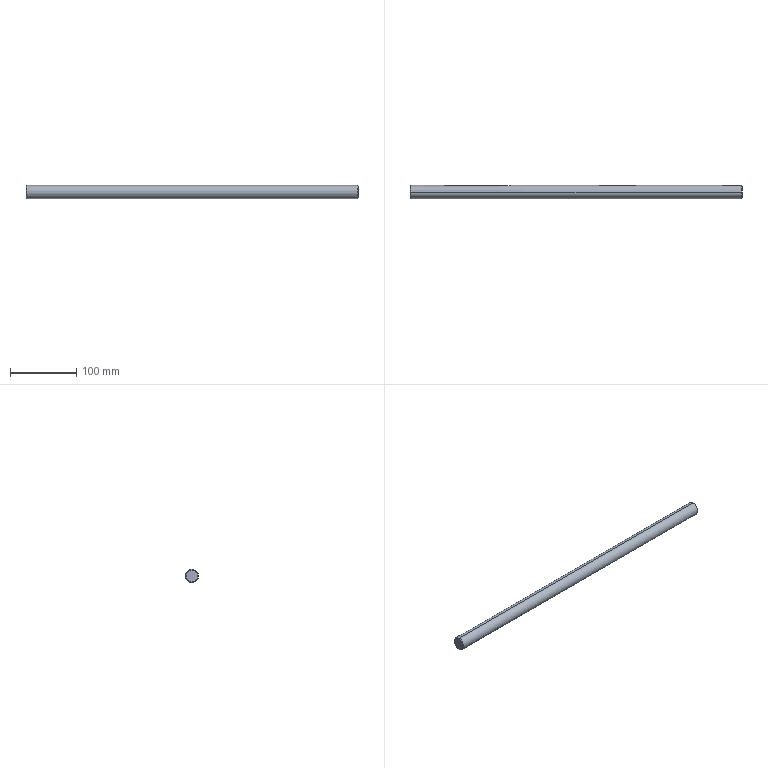Component | SolidWorks | ZL-11-08DriveShaft1-1 | 1 solid | 25 faces | box 503 x 20 x 20 mm | volume 154270 mm3 | plane 11 | cylinder 9 | cone 5 | commonest cylinder face diameters 6 x7 20 x2
build123d program:
from build123d import *

# Parameters (mm, degrees)
SKETCH1_R          = 10
EXTRUDE1_DEPTH     = 251.5
CUT_EXTRUDE1_DEPTH = 3.5
CHAMFER1_SIZE      = 1


with BuildPart() as part:
    # Sketch1 → Extrude1 (new, symmetric)
    with BuildSketch(Plane.XY):
        Circle(SKETCH1_R)
    extrude(amount=EXTRUDE1_DEPTH, both=True)

    # Sketch2 → Cut-Extrude1 (cut)
    with BuildSketch(Plane(origin=(0, 10, 0), x_dir=(-1, 0, 0), z_dir=(0, 1, 0))):
        with BuildLine():
            Line((-3, 251.5), (3, 251.5))
            Line((3, 251.5), (3, 224.5))
            ThreePointArc((3, 224.5), (0, 221.5), (-3, 224.5))
            Line((-3, 224.5), (-3, 251.5))
        make_face()
        with BuildLine():
            Line((-3, -101.5), (-3, -196.5))
            ThreePointArc((-3, -196.5), (0, -199.5), (3, -196.5))
            Line((3, -196.5), (3, -101.5))
            ThreePointArc((3, -101.5), (0, -98.5), (-3, -101.5))
        make_face()
        with BuildLine():
            Line((-3, 88.5), (-3, 38.5))
            ThreePointArc((-3, 38.5), (0, 35.5), (3, 38.5))
            Line((3, 38.5), (3, 88.5))
            ThreePointArc((3, 88.5), (0, 91.5), (-3, 88.5))
        make_face()
    extrude(amount=-CUT_EXTRUDE1_DEPTH, mode=Mode.SUBTRACT)

    # Chamfer1
    chamfer1_edges = [part.edges().sort_by_distance(p)[0] for p in [
        (-10, 0, -251.5),
        (-5.916, -8.062, 251.5),
    ]]
    chamfer(chamfer1_edges, length=CHAMFER1_SIZE)


solid = part.part

# Placed as in the assembly
solid = solid.moved(Location((31.752, 111.22, 0), (0, 90, 0)))
STEP:
#1=COLOUR_RGB('',0.7922,0.8196,0.9333);
#2=FILL_AREA_STYLE_COLOUR('',#1);
#3=FILL_AREA_STYLE('',(#2));
#4=SURFACE_STYLE_FILL_AREA(#3);
#5=SURFACE_SIDE_STYLE('',(#4));
#6=SURFACE_STYLE_USAGE(.BOTH.,#5);
#7=PRESENTATION_STYLE_ASSIGNMENT((#6));
#8=CARTESIAN_POINT('',(-8.651,4.379,0.3543));
#9=VERTEX_POINT('',#8);
#10=CARTESIAN_POINT('',(-8.651,4.379,-0.3543));
#11=VERTEX_POINT('',#10);
#12=CARTESIAN_POINT('',(-8.651,4.379,0.));
#13=DIRECTION('',(-1.,-0.,0.));
#14=DIRECTION('',(0.,0.,-1.));
#15=AXIS2_PLACEMENT_3D('',#12,#13,#14);
#16=CIRCLE('',#15,0.3543);
#17=EDGE_CURVE('',#9,#11,#16,.T.);
#18=ORIENTED_EDGE('',*,*,#17,.F.);
#19=CARTESIAN_POINT('',(-8.612,4.379,0.3937));
#20=VERTEX_POINT('',#19);
#21=CARTESIAN_POINT('',(-8.612,4.379,0.3937));
#22=DIRECTION('',(0.7071,0.,0.7071));
#23=VECTOR('',#22,39.37);
#24=LINE('',#21,#23);
#25=EDGE_CURVE('',#9,#20,#24,.T.);
#26=ORIENTED_EDGE('',*,*,#25,.T.);
#27=CARTESIAN_POINT('',(-8.612,4.379,-0.3937));
#28=VERTEX_POINT('',#27);
#29=CARTESIAN_POINT('',(-8.612,4.379,0.));
#30=DIRECTION('',(1.,0.,-0.));
#31=DIRECTION('',(0.,0.,-1.));
#32=AXIS2_PLACEMENT_3D('',#29,#30,#31);
#33=CIRCLE('',#32,0.3937);
#34=EDGE_CURVE('',#28,#20,#33,.T.);
#35=ORIENTED_EDGE('',*,*,#34,.F.);
#36=CARTESIAN_POINT('',(-8.612,4.379,-0.3937));
#37=DIRECTION('',(0.7071,0.,-0.7071));
#38=VECTOR('',#37,39.37);
#39=LINE('',#36,#38);
#40=EDGE_CURVE('',#11,#28,#39,.T.);
#41=ORIENTED_EDGE('',*,*,#40,.F.);
#42=EDGE_LOOP('',(#18,#26,#35,#41));
#43=FACE_OUTER_BOUND('',#42,.T.);
#44=CARTESIAN_POINT('',(-8.612,4.379,0.));
#45=DIRECTION('',(1.,0.,-0.));
#46=DIRECTION('',(0.,0.,-1.));
#47=AXIS2_PLACEMENT_3D('',#44,#45,#46);
#48=CONICAL_SURFACE('',#47,0.3937,0.7854);
#49=ADVANCED_FACE('',(#43),#48,.T.);
#50=CARTESIAN_POINT('',(11.152,4.379,-0.3543));
#51=VERTEX_POINT('',#50);
#52=CARTESIAN_POINT('',(11.152,4.713,-0.1181));
#53=VERTEX_POINT('',#52);
#54=CARTESIAN_POINT('',(11.152,4.379,0.));
#55=DIRECTION('',(1.,0.,-0.));
#56=DIRECTION('',(0.,0.,-1.));
#57=AXIS2_PLACEMENT_3D('',#54,#55,#56);
#58=CIRCLE('',#57,0.3543);
#59=EDGE_CURVE('',#51,#53,#58,.T.);
#60=ORIENTED_EDGE('',*,*,#59,.F.);
#61=CARTESIAN_POINT('',(11.112,4.379,-0.3937));
#62=VERTEX_POINT('',#61);
#63=CARTESIAN_POINT('',(11.152,4.379,-0.3543));
#64=DIRECTION('',(-0.7071,-0.,-0.7071));
#65=VECTOR('',#64,39.37);
#66=LINE('',#63,#65);
#67=EDGE_CURVE('',#51,#62,#66,.T.);
#68=ORIENTED_EDGE('',*,*,#67,.T.);
#69=CARTESIAN_POINT('',(11.112,4.754,-0.1181));
#70=VERTEX_POINT('',#69);
#71=CARTESIAN_POINT('',(11.112,4.379,0.));
#72=DIRECTION('',(-1.,-0.,0.));
#73=DIRECTION('',(0.,0.,-1.));
#74=AXIS2_PLACEMENT_3D('',#71,#72,#73);
#75=CIRCLE('',#74,0.3937);
#76=EDGE_CURVE('',#70,#62,#75,.T.);
#77=ORIENTED_EDGE('',*,*,#76,.F.);
#78=CARTESIAN_POINT('',(11.152,4.713,-0.1181));
#79=CARTESIAN_POINT('',(11.139,4.727,-0.1181));
#80=CARTESIAN_POINT('',(11.125,4.74,-0.1181));
#81=CARTESIAN_POINT('',(11.112,4.754,-0.1181));
#82=B_SPLINE_CURVE_WITH_KNOTS('',3,(#78,#79,#80,#81),.UNSPECIFIED.,.F.,.F.,(4,4),(0.,0.001453),.UNSPECIFIED.);
#83=EDGE_CURVE('',#53,#70,#82,.T.);
#84=ORIENTED_EDGE('',*,*,#83,.F.);
#85=EDGE_LOOP('',(#60,#68,#77,#84));
#86=FACE_OUTER_BOUND('',#85,.T.);
#87=CARTESIAN_POINT('',(11.152,4.379,0.));
#88=DIRECTION('',(-1.,-0.,0.));
#89=DIRECTION('',(0.,0.,1.));
#90=AXIS2_PLACEMENT_3D('',#87,#88,#89);
#91=CONICAL_SURFACE('',#90,0.3543,0.7854);
#92=ADVANCED_FACE('',(#86),#91,.T.);
#93=ORIENTED_EDGE('',*,*,#67,.F.);
#94=CARTESIAN_POINT('',(11.152,4.379,0.3543));
#95=VERTEX_POINT('',#94);
#96=CARTESIAN_POINT('',(11.152,4.379,0.));
#97=DIRECTION('',(1.,0.,-0.));
#98=DIRECTION('',(0.,0.,-1.));
#99=AXIS2_PLACEMENT_3D('',#96,#97,#98);
#100=CIRCLE('',#99,0.3543);
#101=EDGE_CURVE('',#95,#51,#100,.T.);
#102=ORIENTED_EDGE('',*,*,#101,.F.);
#103=CARTESIAN_POINT('',(11.112,4.379,0.3937));
#104=VERTEX_POINT('',#103);
#105=CARTESIAN_POINT('',(11.152,4.379,0.3543));
#106=DIRECTION('',(-0.7071,-0.,0.7071));
#107=VECTOR('',#106,39.37);
#108=LINE('',#105,#107);
#109=EDGE_CURVE('',#95,#104,#108,.T.);
#110=ORIENTED_EDGE('',*,*,#109,.T.);
#111=CARTESIAN_POINT('',(11.112,4.379,0.));
#112=DIRECTION('',(-1.,-0.,0.));
#113=DIRECTION('',(0.,-0.,-1.));
#114=AXIS2_PLACEMENT_3D('',#111,#112,#113);
#115=CIRCLE('',#114,0.3937);
#116=EDGE_CURVE('',#62,#104,#115,.T.);
#117=ORIENTED_EDGE('',*,*,#116,.F.);
#118=EDGE_LOOP('',(#93,#102,#110,#117));
#119=FACE_OUTER_BOUND('',#118,.T.);
#120=CARTESIAN_POINT('',(11.152,4.379,0.));
#121=DIRECTION('',(-1.,-0.,0.));
#122=DIRECTION('',(0.,0.,1.));
#123=AXIS2_PLACEMENT_3D('',#120,#121,#122);
#124=CONICAL_SURFACE('',#123,0.3543,0.7854);
#125=ADVANCED_FACE('',(#119),#124,.T.);
#126=CARTESIAN_POINT('',(4.852,4.635,0.));
#127=VERTEX_POINT('',#126);
#128=CARTESIAN_POINT('',(4.734,4.635,-0.1181));
#129=VERTEX_POINT('',#128);
#130=CARTESIAN_POINT('',(4.734,4.635,0.));
#131=DIRECTION('',(-0.,1.,-0.));
#132=DIRECTION('',(1.,0.,-0.));
#133=AXIS2_PLACEMENT_3D('',#130,#131,#132);
#134=CIRCLE('',#133,0.1181);
#135=EDGE_CURVE('',#127,#129,#134,.T.);
#136=ORIENTED_EDGE('',*,*,#135,.F.);
#137=CARTESIAN_POINT('',(4.852,4.772,0.));
#138=VERTEX_POINT('',#137);
#139=CARTESIAN_POINT('',(4.852,4.635,0.));
#140=DIRECTION('',(-0.,1.,-0.));
#141=VECTOR('',#140,39.37);
#142=LINE('',#139,#141);
#143=EDGE_CURVE('',#127,#138,#142,.T.);
#144=ORIENTED_EDGE('',*,*,#143,.T.);
#145=CARTESIAN_POINT('',(4.734,4.754,-0.1181));
#146=VERTEX_POINT('',#145);
#147=CARTESIAN_POINT('',(4.734,4.754,-0.1181));
#148=CARTESIAN_POINT('',(4.742,4.754,-0.1181));
#149=CARTESIAN_POINT('',(4.75,4.755,-0.1173));
#150=CARTESIAN_POINT('',(4.765,4.755,-0.1143));
#151=CARTESIAN_POINT('',(4.773,4.756,-0.112));
#152=CARTESIAN_POINT('',(4.794,4.759,-0.1031));
#153=CARTESIAN_POINT('',(4.807,4.761,-0.09437));
#154=CARTESIAN_POINT('',(4.823,4.765,-0.07814));
#155=CARTESIAN_POINT('',(4.828,4.766,-0.07211));
#156=CARTESIAN_POINT('',(4.837,4.768,-0.05931));
#157=CARTESIAN_POINT('',(4.84,4.769,-0.05255));
#158=CARTESIAN_POINT('',(4.846,4.771,-0.03831));
#159=CARTESIAN_POINT('',(4.849,4.771,-0.03076));
#160=CARTESIAN_POINT('',(4.852,4.772,-0.01557));
#161=CARTESIAN_POINT('',(4.852,4.772,-0.00785));
#162=CARTESIAN_POINT('',(4.852,4.772,0.));
#163=B_SPLINE_CURVE_WITH_KNOTS('',3,(#147,#148,#149,#150,#151,#152,#153,#154,#155,#156,#157,#158,#159,#160,#161,#162),.UNSPECIFIED.,.F.,.F.,(4,2,2,2,2,2,2,4),(0.01415,0.01474,0.01533,0.01651,0.0171,0.01769,0.01828,0.01887),.UNSPECIFIED.);
#164=EDGE_CURVE('',#146,#138,#163,.T.);
#165=ORIENTED_EDGE('',*,*,#164,.F.);
#166=CARTESIAN_POINT('',(4.734,4.635,-0.1181));
#167=DIRECTION('',(-0.,1.,-0.));
#168=VECTOR('',#167,39.37);
#169=LINE('',#166,#168);
#170=EDGE_CURVE('',#129,#146,#169,.T.);
#171=ORIENTED_EDGE('',*,*,#170,.F.);
#172=EDGE_LOOP('',(#136,#144,#165,#171));
#173=FACE_OUTER_BOUND('',#172,.T.);
#174=CARTESIAN_POINT('',(4.734,4.635,0.));
#175=DIRECTION('',(-0.,1.,-0.));
#176=DIRECTION('',(1.,0.,-0.));
#177=AXIS2_PLACEMENT_3D('',#174,#175,#176);
#178=CYLINDRICAL_SURFACE('',#177,0.1181);
#179=ADVANCED_FACE('',(#173),#178,.F.);
#180=CARTESIAN_POINT('',(-2.628,4.635,0.));
#181=VERTEX_POINT('',#180);
#182=CARTESIAN_POINT('',(-2.746,4.635,-0.1181));
#183=VERTEX_POINT('',#182);
#184=CARTESIAN_POINT('',(-2.746,4.635,0.));
#185=DIRECTION('',(-0.,1.,-0.));
#186=DIRECTION('',(1.,0.,-0.));
#187=AXIS2_PLACEMENT_3D('',#184,#185,#186);
#188=CIRCLE('',#187,0.1181);
#189=EDGE_CURVE('',#181,#183,#188,.T.);
#190=ORIENTED_EDGE('',*,*,#189,.F.);
#191=CARTESIAN_POINT('',(-2.628,4.772,0.));
#192=VERTEX_POINT('',#191);
#193=CARTESIAN_POINT('',(-2.628,4.635,0.));
#194=DIRECTION('',(-0.,1.,-0.));
#195=VECTOR('',#194,39.37);
#196=LINE('',#193,#195);
#197=EDGE_CURVE('',#181,#192,#196,.T.);
#198=ORIENTED_EDGE('',*,*,#197,.T.);
#199=CARTESIAN_POINT('',(-2.746,4.754,-0.1181));
#200=VERTEX_POINT('',#199);
#201=CARTESIAN_POINT('',(-2.746,4.754,-0.1181));
#202=CARTESIAN_POINT('',(-2.738,4.754,-0.1181));
#203=CARTESIAN_POINT('',(-2.731,4.755,-0.1173));
#204=CARTESIAN_POINT('',(-2.715,4.755,-0.1143));
#205=CARTESIAN_POINT('',(-2.708,4.756,-0.112));
#206=CARTESIAN_POINT('',(-2.686,4.759,-0.1031));
#207=CARTESIAN_POINT('',(-2.673,4.761,-0.09437));
#208=CARTESIAN_POINT('',(-2.657,4.765,-0.07814));
#209=CARTESIAN_POINT('',(-2.652,4.766,-0.07211));
#210=CARTESIAN_POINT('',(-2.644,4.768,-0.05931));
#211=CARTESIAN_POINT('',(-2.64,4.769,-0.05255));
#212=CARTESIAN_POINT('',(-2.634,4.771,-0.03831));
#213=CARTESIAN_POINT('',(-2.632,4.771,-0.03076));
#214=CARTESIAN_POINT('',(-2.629,4.772,-0.01557));
#215=CARTESIAN_POINT('',(-2.628,4.772,-0.00785));
#216=CARTESIAN_POINT('',(-2.628,4.772,0.));
#217=B_SPLINE_CURVE_WITH_KNOTS('',3,(#201,#202,#203,#204,#205,#206,#207,#208,#209,#210,#211,#212,#213,#214,#215,#216),.UNSPECIFIED.,.F.,.F.,(4,2,2,2,2,2,2,4),(0.01415,0.01474,0.01533,0.01651,0.0171,0.01769,0.01828,0.01887),.UNSPECIFIED.);
#218=EDGE_CURVE('',#200,#192,#217,.T.);
#219=ORIENTED_EDGE('',*,*,#218,.F.);
#220=CARTESIAN_POINT('',(-2.746,4.635,-0.1181));
#221=DIRECTION('',(-0.,1.,-0.));
#222=VECTOR('',#221,39.37);
#223=LINE('',#220,#222);
#224=EDGE_CURVE('',#183,#200,#223,.T.);
#225=ORIENTED_EDGE('',*,*,#224,.F.);
#226=EDGE_LOOP('',(#190,#198,#219,#225));
#227=FACE_OUTER_BOUND('',#226,.T.);
#228=CARTESIAN_POINT('',(-2.746,4.635,0.));
#229=DIRECTION('',(-0.,1.,-0.));
#230=DIRECTION('',(1.,0.,-0.));
#231=AXIS2_PLACEMENT_3D('',#228,#229,#230);
#232=CYLINDRICAL_SURFACE('',#231,0.1181);
#233=ADVANCED_FACE('',(#227),#232,.F.);
#234=ORIENTED_EDGE('',*,*,#164,.T.);
#235=CARTESIAN_POINT('',(4.734,4.754,0.1181));
#236=VERTEX_POINT('',#235);
#237=CARTESIAN_POINT('',(4.852,4.772,0.));
#238=CARTESIAN_POINT('',(4.852,4.772,0.007855));
#239=CARTESIAN_POINT('',(4.852,4.772,0.01557));
#240=CARTESIAN_POINT('',(4.849,4.771,0.03073));
#241=CARTESIAN_POINT('',(4.846,4.771,0.03826));
#242=CARTESIAN_POINT('',(4.84,4.769,0.05255));
#243=CARTESIAN_POINT('',(4.837,4.768,0.05932));
#244=CARTESIAN_POINT('',(4.828,4.766,0.07213));
#245=CARTESIAN_POINT('',(4.823,4.765,0.07815));
#246=CARTESIAN_POINT('',(4.807,4.761,0.09439));
#247=CARTESIAN_POINT('',(4.794,4.759,0.1032));
#248=CARTESIAN_POINT('',(4.773,4.756,0.112));
#249=CARTESIAN_POINT('',(4.765,4.755,0.1143));
#250=CARTESIAN_POINT('',(4.75,4.755,0.1174));
#251=CARTESIAN_POINT('',(4.742,4.754,0.1181));
#252=CARTESIAN_POINT('',(4.734,4.754,0.1181));
#253=B_SPLINE_CURVE_WITH_KNOTS('',3,(#237,#238,#239,#240,#241,#242,#243,#244,#245,#246,#247,#248,#249,#250,#251,#252),.UNSPECIFIED.,.F.,.F.,(4,2,2,2,2,2,2,4),(0.,0.0005898,0.00118,0.001769,0.002359,0.003539,0.004129,0.004718),.UNSPECIFIED.);
#254=EDGE_CURVE('',#138,#236,#253,.T.);
#255=ORIENTED_EDGE('',*,*,#254,.T.);
#256=CARTESIAN_POINT('',(2.766,4.754,0.1181));
#257=VERTEX_POINT('',#256);
#258=CARTESIAN_POINT('',(11.152,4.754,0.1181));
#259=DIRECTION('',(-1.,-0.,0.));
#260=VECTOR('',#259,39.37);
#261=LINE('',#258,#260);
#262=EDGE_CURVE('',#236,#257,#261,.T.);
#263=ORIENTED_EDGE('',*,*,#262,.T.);
#264=CARTESIAN_POINT('',(2.766,4.754,-0.1181));
#265=VERTEX_POINT('',#264);
#266=CARTESIAN_POINT('',(2.766,4.754,0.1181));
#267=CARTESIAN_POINT('',(2.758,4.754,0.1181));
#268=CARTESIAN_POINT('',(2.75,4.755,0.1173));
#269=CARTESIAN_POINT('',(2.735,4.755,0.1143));
#270=CARTESIAN_POINT('',(2.728,4.756,0.112));
#271=CARTESIAN_POINT('',(2.713,4.758,0.1061));
#272=CARTESIAN_POINT('',(2.706,4.759,0.1024));
#273=CARTESIAN_POINT('',(2.694,4.761,0.09385));
#274=CARTESIAN_POINT('',(2.688,4.762,0.08892));
#275=CARTESIAN_POINT('',(2.677,4.765,0.07802));
#276=CARTESIAN_POINT('',(2.672,4.766,0.0721));
#277=CARTESIAN_POINT('',(2.663,4.768,0.05934));
#278=CARTESIAN_POINT('',(2.66,4.769,0.05242));
#279=CARTESIAN_POINT('',(2.654,4.771,0.03819));
#280=CARTESIAN_POINT('',(2.652,4.771,0.03082));
#281=CARTESIAN_POINT('',(2.648,4.772,0.01556));
#282=CARTESIAN_POINT('',(2.648,4.772,0.007729));
#283=CARTESIAN_POINT('',(2.648,4.772,-0.007742));
#284=CARTESIAN_POINT('',(2.648,4.772,-0.0155));
#285=CARTESIAN_POINT('',(2.652,4.771,-0.03083));
#286=CARTESIAN_POINT('',(2.654,4.771,-0.03822));
#287=CARTESIAN_POINT('',(2.66,4.769,-0.05246));
#288=CARTESIAN_POINT('',(2.663,4.768,-0.05937));
#289=CARTESIAN_POINT('',(2.672,4.766,-0.07215));
#290=CARTESIAN_POINT('',(2.677,4.765,-0.07806));
#291=CARTESIAN_POINT('',(2.688,4.762,-0.08896));
#292=CARTESIAN_POINT('',(2.694,4.761,-0.09389));
#293=CARTESIAN_POINT('',(2.706,4.759,-0.1024));
#294=CARTESIAN_POINT('',(2.713,4.758,-0.1061));
#295=CARTESIAN_POINT('',(2.728,4.756,-0.112));
#296=CARTESIAN_POINT('',(2.735,4.755,-0.1143));
#297=CARTESIAN_POINT('',(2.75,4.755,-0.1173));
#298=CARTESIAN_POINT('',(2.758,4.754,-0.1181));
#299=CARTESIAN_POINT('',(2.766,4.754,-0.1181));
#300=B_SPLINE_CURVE_WITH_KNOTS('',3,(#266,#267,#268,#269,#270,#271,#272,#273,#274,#275,#276,#277,#278,#279,#280,#281,#282,#283,#284,#285,#286,#287,#288,#289,#290,#291,#292,#293,#294,#295,#296,#297,#298,#299),.UNSPECIFIED.,.F.,.F.,(4,2,2,2,2,2,2,2,2,2,2,2,2,2,2,2,4),(0.004718,0.005308,0.005897,0.006487,0.007076,0.007666,0.008255,0.008845,0.009434,0.01002,0.01061,0.0112,0.01179,0.01238,0.01297,0.01356,0.01415),.UNSPECIFIED.);
#301=EDGE_CURVE('',#257,#265,#300,.T.);
#302=ORIENTED_EDGE('',*,*,#301,.T.);
#303=CARTESIAN_POINT('',(11.152,4.754,-0.1181));
#304=DIRECTION('',(1.,0.,-0.));
#305=VECTOR('',#304,39.37);
#306=LINE('',#303,#305);
#307=EDGE_CURVE('',#265,#146,#306,.T.);
#308=ORIENTED_EDGE('',*,*,#307,.T.);
#309=EDGE_LOOP('',(#234,#255,#263,#302,#308));
#310=FACE_BOUND('',#309,.T.);
#311=ORIENTED_EDGE('',*,*,#218,.T.);
#312=CARTESIAN_POINT('',(-2.746,4.754,0.1181));
#313=VERTEX_POINT('',#312);
#314=CARTESIAN_POINT('',(-2.628,4.772,0.));
#315=CARTESIAN_POINT('',(-2.628,4.772,0.007855));
#316=CARTESIAN_POINT('',(-2.629,4.772,0.01557));
#317=CARTESIAN_POINT('',(-2.632,4.771,0.03073));
#318=CARTESIAN_POINT('',(-2.634,4.771,0.03826));
#319=CARTESIAN_POINT('',(-2.64,4.769,0.05255));
#320=CARTESIAN_POINT('',(-2.644,4.768,0.05932));
#321=CARTESIAN_POINT('',(-2.652,4.766,0.07213));
#322=CARTESIAN_POINT('',(-2.657,4.765,0.07815));
#323=CARTESIAN_POINT('',(-2.673,4.761,0.09439));
#324=CARTESIAN_POINT('',(-2.686,4.759,0.1032));
#325=CARTESIAN_POINT('',(-2.708,4.756,0.112));
#326=CARTESIAN_POINT('',(-2.715,4.755,0.1143));
#327=CARTESIAN_POINT('',(-2.731,4.755,0.1174));
#328=CARTESIAN_POINT('',(-2.738,4.754,0.1181));
#329=CARTESIAN_POINT('',(-2.746,4.754,0.1181));
#330=B_SPLINE_CURVE_WITH_KNOTS('',3,(#314,#315,#316,#317,#318,#319,#320,#321,#322,#323,#324,#325,#326,#327,#328,#329),.UNSPECIFIED.,.F.,.F.,(4,2,2,2,2,2,2,4),(0.,0.0005898,0.00118,0.001769,0.002359,0.003539,0.004129,0.004718),.UNSPECIFIED.);
#331=EDGE_CURVE('',#192,#313,#330,.T.);
#332=ORIENTED_EDGE('',*,*,#331,.T.);
#333=CARTESIAN_POINT('',(-6.486,4.754,0.1181));
#334=VERTEX_POINT('',#333);
#335=CARTESIAN_POINT('',(11.152,4.754,0.1181));
#336=DIRECTION('',(-1.,-0.,0.));
#337=VECTOR('',#336,39.37);
#338=LINE('',#335,#337);
#339=EDGE_CURVE('',#313,#334,#338,.T.);
#340=ORIENTED_EDGE('',*,*,#339,.T.);
#341=CARTESIAN_POINT('',(-6.486,4.754,-0.1181));
#342=VERTEX_POINT('',#341);
#343=CARTESIAN_POINT('',(-6.486,4.754,0.1181));
#344=CARTESIAN_POINT('',(-6.494,4.754,0.1181));
#345=CARTESIAN_POINT('',(-6.502,4.755,0.1173));
#346=CARTESIAN_POINT('',(-6.517,4.755,0.1143));
#347=CARTESIAN_POINT('',(-6.524,4.756,0.112));
#348=CARTESIAN_POINT('',(-6.539,4.758,0.1061));
#349=CARTESIAN_POINT('',(-6.546,4.759,0.1024));
#350=CARTESIAN_POINT('',(-6.558,4.761,0.09385));
#351=CARTESIAN_POINT('',(-6.564,4.762,0.08892));
#352=CARTESIAN_POINT('',(-6.575,4.765,0.07802));
#353=CARTESIAN_POINT('',(-6.58,4.766,0.0721));
#354=CARTESIAN_POINT('',(-6.589,4.768,0.05934));
#355=CARTESIAN_POINT('',(-6.592,4.769,0.05242));
#356=CARTESIAN_POINT('',(-6.598,4.771,0.03819));
#357=CARTESIAN_POINT('',(-6.6,4.771,0.03082));
#358=CARTESIAN_POINT('',(-6.603,4.772,0.01556));
#359=CARTESIAN_POINT('',(-6.604,4.772,0.007729));
#360=CARTESIAN_POINT('',(-6.604,4.772,-0.007742));
#361=CARTESIAN_POINT('',(-6.603,4.772,-0.0155));
#362=CARTESIAN_POINT('',(-6.6,4.771,-0.03083));
#363=CARTESIAN_POINT('',(-6.598,4.771,-0.03822));
#364=CARTESIAN_POINT('',(-6.592,4.769,-0.05246));
#365=CARTESIAN_POINT('',(-6.589,4.768,-0.05937));
#366=CARTESIAN_POINT('',(-6.58,4.766,-0.07215));
#367=CARTESIAN_POINT('',(-6.575,4.765,-0.07806));
#368=CARTESIAN_POINT('',(-6.564,4.762,-0.08896));
#369=CARTESIAN_POINT('',(-6.558,4.761,-0.09389));
#370=CARTESIAN_POINT('',(-6.545,4.759,-0.1024));
#371=CARTESIAN_POINT('',(-6.539,4.758,-0.1061));
#372=CARTESIAN_POINT('',(-6.524,4.756,-0.112));
#373=CARTESIAN_POINT('',(-6.517,4.755,-0.1143));
#374=CARTESIAN_POINT('',(-6.502,4.755,-0.1173));
#375=CARTESIAN_POINT('',(-6.494,4.754,-0.1181));
#376=CARTESIAN_POINT('',(-6.486,4.754,-0.1181));
#377=B_SPLINE_CURVE_WITH_KNOTS('',3,(#343,#344,#345,#346,#347,#348,#349,#350,#351,#352,#353,#354,#355,#356,#357,#358,#359,#360,#361,#362,#363,#364,#365,#366,#367,#368,#369,#370,#371,#372,#373,#374,#375,#376),.UNSPECIFIED.,.F.,.F.,(4,2,2,2,2,2,2,2,2,2,2,2,2,2,2,2,4),(0.004718,0.005308,0.005897,0.006487,0.007076,0.007666,0.008255,0.008845,0.009434,0.01002,0.01061,0.0112,0.01179,0.01238,0.01297,0.01356,0.01415),.UNSPECIFIED.);
#378=EDGE_CURVE('',#334,#342,#377,.T.);
#379=ORIENTED_EDGE('',*,*,#378,.T.);
#380=CARTESIAN_POINT('',(11.152,4.754,-0.1181));
#381=DIRECTION('',(1.,0.,-0.));
#382=VECTOR('',#381,39.37);
#383=LINE('',#380,#382);
#384=EDGE_CURVE('',#342,#200,#383,.T.);
#385=ORIENTED_EDGE('',*,*,#384,.T.);
#386=EDGE_LOOP('',(#311,#332,#340,#379,#385));
#387=FACE_BOUND('',#386,.T.);
#388=ORIENTED_EDGE('',*,*,#76,.T.);
#389=CARTESIAN_POINT('',(11.152,4.379,-0.3937));
#390=DIRECTION('',(-1.,-0.,0.));
#391=VECTOR('',#390,39.37);
#392=LINE('',#389,#391);
#393=EDGE_CURVE('',#62,#28,#392,.T.);
#394=ORIENTED_EDGE('',*,*,#393,.T.);
#395=ORIENTED_EDGE('',*,*,#34,.T.);
#396=CARTESIAN_POINT('',(11.152,4.379,0.3937));
#397=DIRECTION('',(-1.,-0.,0.));
#398=VECTOR('',#397,39.37);
#399=LINE('',#396,#398);
#400=EDGE_CURVE('',#104,#20,#399,.T.);
#401=ORIENTED_EDGE('',*,*,#400,.F.);
#402=CARTESIAN_POINT('',(11.112,4.754,0.1181));
#403=VERTEX_POINT('',#402);
#404=CARTESIAN_POINT('',(11.112,4.379,0.));
#405=DIRECTION('',(-1.,-0.,0.));
#406=DIRECTION('',(0.,0.,-1.));
#407=AXIS2_PLACEMENT_3D('',#404,#405,#406);
#408=CIRCLE('',#407,0.3937);
#409=EDGE_CURVE('',#104,#403,#408,.T.);
#410=ORIENTED_EDGE('',*,*,#409,.T.);
#411=CARTESIAN_POINT('',(10.089,4.754,0.1181));
#412=VERTEX_POINT('',#411);
#413=CARTESIAN_POINT('',(11.152,4.754,0.1181));
#414=DIRECTION('',(-1.,-0.,0.));
#415=VECTOR('',#414,39.37);
#416=LINE('',#413,#415);
#417=EDGE_CURVE('',#403,#412,#416,.T.);
#418=ORIENTED_EDGE('',*,*,#417,.T.);
#419=CARTESIAN_POINT('',(10.089,4.754,-0.1181));
#420=VERTEX_POINT('',#419);
#421=CARTESIAN_POINT('',(10.089,4.754,0.1181));
#422=CARTESIAN_POINT('',(10.081,4.754,0.1181));
#423=CARTESIAN_POINT('',(10.073,4.755,0.1173));
#424=CARTESIAN_POINT('',(10.058,4.755,0.1143));
#425=CARTESIAN_POINT('',(10.05,4.756,0.112));
#426=CARTESIAN_POINT('',(10.036,4.758,0.1061));
#427=CARTESIAN_POINT('',(10.029,4.759,0.1024));
#428=CARTESIAN_POINT('',(10.017,4.761,0.09389));
#429=CARTESIAN_POINT('',(10.011,4.762,0.08893));
#430=CARTESIAN_POINT('',(9.994,4.766,0.0727));
#431=CARTESIAN_POINT('',(9.986,4.768,0.0596));
#432=CARTESIAN_POINT('',(9.977,4.771,0.03832));
#433=CARTESIAN_POINT('',(9.974,4.771,0.03083));
#434=CARTESIAN_POINT('',(9.971,4.772,0.01556));
#435=CARTESIAN_POINT('',(9.971,4.772,0.007869));
#436=CARTESIAN_POINT('',(9.971,4.772,-0.007636));
#437=CARTESIAN_POINT('',(9.971,4.772,-0.01551));
#438=CARTESIAN_POINT('',(9.974,4.771,-0.0307));
#439=CARTESIAN_POINT('',(9.977,4.771,-0.03808));
#440=CARTESIAN_POINT('',(9.983,4.769,-0.05244));
#441=CARTESIAN_POINT('',(9.986,4.768,-0.05928));
#442=CARTESIAN_POINT('',(9.995,4.766,-0.07203));
#443=CARTESIAN_POINT('',(10.,4.765,-0.07804));
#444=CARTESIAN_POINT('',(10.011,4.762,-0.08894));
#445=CARTESIAN_POINT('',(10.016,4.761,-0.0938));
#446=CARTESIAN_POINT('',(10.029,4.759,-0.1024));
#447=CARTESIAN_POINT('',(10.036,4.758,-0.1061));
#448=CARTESIAN_POINT('',(10.05,4.756,-0.112));
#449=CARTESIAN_POINT('',(10.058,4.755,-0.1142));
#450=CARTESIAN_POINT('',(10.073,4.755,-0.1173));
#451=CARTESIAN_POINT('',(10.081,4.754,-0.1181));
#452=CARTESIAN_POINT('',(10.089,4.754,-0.1181));
#453=B_SPLINE_CURVE_WITH_KNOTS('',3,(#421,#422,#423,#424,#425,#426,#427,#428,#429,#430,#431,#432,#433,#434,#435,#436,#437,#438,#439,#440,#441,#442,#443,#444,#445,#446,#447,#448,#449,#450,#451,#452),.UNSPECIFIED.,.F.,.F.,(4,2,2,2,2,2,2,2,2,2,2,2,2,2,2,4),(0.,0.0005894,0.001179,0.001768,0.002358,0.003536,0.004126,0.004715,0.005305,0.005894,0.006484,0.007073,0.007662,0.008252,0.008841,0.009431),.UNSPECIFIED.);
#454=EDGE_CURVE('',#412,#420,#453,.T.);
#455=ORIENTED_EDGE('',*,*,#454,.T.);
#456=CARTESIAN_POINT('',(11.152,4.754,-0.1181));
#457=DIRECTION('',(1.,0.,-0.));
#458=VECTOR('',#457,39.37);
#459=LINE('',#456,#458);
#460=EDGE_CURVE('',#420,#70,#459,.T.);
#461=ORIENTED_EDGE('',*,*,#460,.T.);
#462=EDGE_LOOP('',(#388,#394,#395,#401,#410,#418,#455,#461));
#463=FACE_OUTER_BOUND('',#462,.T.);
#464=CARTESIAN_POINT('',(11.152,4.379,0.));
#465=DIRECTION('',(-1.,-0.,0.));
#466=DIRECTION('',(0.,0.,1.));
#467=AXIS2_PLACEMENT_3D('',#464,#465,#466);
#468=CYLINDRICAL_SURFACE('',#467,0.3937);
#469=ADVANCED_FACE('',(#310,#387,#463),#468,.T.);
#470=ORIENTED_EDGE('',*,*,#393,.F.);
#471=ORIENTED_EDGE('',*,*,#116,.T.);
#472=ORIENTED_EDGE('',*,*,#400,.T.);
#473=CARTESIAN_POINT('',(-8.612,4.379,0.));
#474=DIRECTION('',(1.,0.,-0.));
#475=DIRECTION('',(0.,0.,-1.));
#476=AXIS2_PLACEMENT_3D('',#473,#474,#475);
#477=CIRCLE('',#476,0.3937);
#478=EDGE_CURVE('',#20,#28,#477,.T.);
#479=ORIENTED_EDGE('',*,*,#478,.T.);
#480=EDGE_LOOP('',(#470,#471,#472,#479));
#481=FACE_OUTER_BOUND('',#480,.T.);
#482=CARTESIAN_POINT('',(11.152,4.379,0.));
#483=DIRECTION('',(-1.,-0.,0.));
#484=DIRECTION('',(0.,0.,1.));
#485=AXIS2_PLACEMENT_3D('',#482,#483,#484);
#486=CYLINDRICAL_SURFACE('',#485,0.3937);
#487=ADVANCED_FACE('',(#481),#486,.T.);
#488=CARTESIAN_POINT('',(11.152,4.635,0.1181));
#489=VERTEX_POINT('',#488);
#490=CARTESIAN_POINT('',(11.152,4.713,0.1181));
#491=VERTEX_POINT('',#490);
#492=CARTESIAN_POINT('',(11.152,4.635,0.1181));
#493=DIRECTION('',(-0.,1.,-0.));
#494=VECTOR('',#493,39.37);
#495=LINE('',#492,#494);
#496=EDGE_CURVE('',#489,#491,#495,.T.);
#497=ORIENTED_EDGE('',*,*,#496,.T.);
#498=CARTESIAN_POINT('',(11.152,4.379,0.));
#499=DIRECTION('',(1.,0.,-0.));
#500=DIRECTION('',(0.,0.,-1.));
#501=AXIS2_PLACEMENT_3D('',#498,#499,#500);
#502=CIRCLE('',#501,0.3543);
#503=EDGE_CURVE('',#491,#95,#502,.T.);
#504=ORIENTED_EDGE('',*,*,#503,.T.);
#505=ORIENTED_EDGE('',*,*,#101,.T.);
#506=ORIENTED_EDGE('',*,*,#59,.T.);
#507=CARTESIAN_POINT('',(11.152,4.635,-0.1181));
#508=VERTEX_POINT('',#507);
#509=CARTESIAN_POINT('',(11.152,4.635,-0.1181));
#510=DIRECTION('',(-0.,1.,-0.));
#511=VECTOR('',#510,39.37);
#512=LINE('',#509,#511);
#513=EDGE_CURVE('',#508,#53,#512,.T.);
#514=ORIENTED_EDGE('',*,*,#513,.F.);
#515=CARTESIAN_POINT('',(11.152,4.635,-0.1181));
#516=DIRECTION('',(-0.,-0.,-1.));
#517=VECTOR('',#516,39.37);
#518=LINE('',#515,#517);
#519=EDGE_CURVE('',#489,#508,#518,.T.);
#520=ORIENTED_EDGE('',*,*,#519,.F.);
#521=EDGE_LOOP('',(#497,#504,#505,#506,#514,#520));
#522=FACE_OUTER_BOUND('',#521,.T.);
#523=CARTESIAN_POINT('',(11.152,4.379,0.));
#524=DIRECTION('',(1.,0.,-0.));
#525=DIRECTION('',(-0.,-0.,-1.));
#526=AXIS2_PLACEMENT_3D('',#523,#524,#525);
#527=PLANE('',#526);
#528=ADVANCED_FACE('',(#522),#527,.T.);
#529=CARTESIAN_POINT('',(-8.651,4.379,0.));
#530=DIRECTION('',(-1.,-0.,0.));
#531=DIRECTION('',(0.,0.,-1.));
#532=AXIS2_PLACEMENT_3D('',#529,#530,#531);
#533=CIRCLE('',#532,0.3543);
#534=EDGE_CURVE('',#11,#9,#533,.T.);
#535=ORIENTED_EDGE('',*,*,#534,.T.);
#536=ORIENTED_EDGE('',*,*,#17,.T.);
#537=EDGE_LOOP('',(#535,#536));
#538=FACE_OUTER_BOUND('',#537,.T.);
#539=CARTESIAN_POINT('',(-8.651,4.379,0.));
#540=DIRECTION('',(1.,0.,-0.));
#541=DIRECTION('',(-0.,-0.,-1.));
#542=AXIS2_PLACEMENT_3D('',#539,#540,#541);
#543=PLANE('',#542);
#544=ADVANCED_FACE('',(#538),#543,.F.);
#545=ORIENTED_EDGE('',*,*,#197,.F.);
#546=CARTESIAN_POINT('',(-2.746,4.635,0.1181));
#547=VERTEX_POINT('',#546);
#548=CARTESIAN_POINT('',(-2.746,4.635,0.));
#549=DIRECTION('',(-0.,1.,-0.));
#550=DIRECTION('',(1.,0.,-0.));
#551=AXIS2_PLACEMENT_3D('',#548,#549,#550);
#552=CIRCLE('',#551,0.1181);
#553=EDGE_CURVE('',#547,#181,#552,.T.);
#554=ORIENTED_EDGE('',*,*,#553,.F.);
#555=CARTESIAN_POINT('',(-2.746,4.635,0.1181));
#556=DIRECTION('',(-0.,1.,-0.));
#557=VECTOR('',#556,39.37);
#558=LINE('',#555,#557);
#559=EDGE_CURVE('',#547,#313,#558,.T.);
#560=ORIENTED_EDGE('',*,*,#559,.T.);
#561=ORIENTED_EDGE('',*,*,#331,.F.);
#562=EDGE_LOOP('',(#545,#554,#560,#561));
#563=FACE_OUTER_BOUND('',#562,.T.);
#564=CARTESIAN_POINT('',(-2.746,4.635,0.));
#565=DIRECTION('',(-0.,1.,-0.));
#566=DIRECTION('',(1.,0.,-0.));
#567=AXIS2_PLACEMENT_3D('',#564,#565,#566);
#568=CYLINDRICAL_SURFACE('',#567,0.1181);
#569=ADVANCED_FACE('',(#563),#568,.F.);
#570=ORIENTED_EDGE('',*,*,#559,.F.);
#571=CARTESIAN_POINT('',(-6.486,4.635,0.1181));
#572=VERTEX_POINT('',#571);
#573=CARTESIAN_POINT('',(-2.746,4.635,0.1181));
#574=DIRECTION('',(1.,0.,-0.));
#575=VECTOR('',#574,39.37);
#576=LINE('',#573,#575);
#577=EDGE_CURVE('',#572,#547,#576,.T.);
#578=ORIENTED_EDGE('',*,*,#577,.F.);
#579=CARTESIAN_POINT('',(-6.486,4.635,0.1181));
#580=DIRECTION('',(-0.,1.,-0.));
#581=VECTOR('',#580,39.37);
#582=LINE('',#579,#581);
#583=EDGE_CURVE('',#572,#334,#582,.T.);
#584=ORIENTED_EDGE('',*,*,#583,.T.);
#585=ORIENTED_EDGE('',*,*,#339,.F.);
#586=EDGE_LOOP('',(#570,#578,#584,#585));
#587=FACE_OUTER_BOUND('',#586,.T.);
#588=CARTESIAN_POINT('',(-2.746,4.635,0.1181));
#589=DIRECTION('',(0.,0.,1.));
#590=DIRECTION('',(1.,0.,-0.));
#591=AXIS2_PLACEMENT_3D('',#588,#589,#590);
#592=PLANE('',#591);
#593=ADVANCED_FACE('',(#587),#592,.F.);
#594=ORIENTED_EDGE('',*,*,#583,.F.);
#595=CARTESIAN_POINT('',(-6.486,4.635,-0.1181));
#596=VERTEX_POINT('',#595);
#597=CARTESIAN_POINT('',(-6.486,4.635,0.));
#598=DIRECTION('',(-0.,1.,-0.));
#599=DIRECTION('',(1.,0.,-0.));
#600=AXIS2_PLACEMENT_3D('',#597,#598,#599);
#601=CIRCLE('',#600,0.1181);
#602=EDGE_CURVE('',#596,#572,#601,.T.);
#603=ORIENTED_EDGE('',*,*,#602,.F.);
#604=CARTESIAN_POINT('',(-6.486,4.635,-0.1181));
#605=DIRECTION('',(-0.,1.,-0.));
#606=VECTOR('',#605,39.37);
#607=LINE('',#604,#606);
#608=EDGE_CURVE('',#596,#342,#607,.T.);
#609=ORIENTED_EDGE('',*,*,#608,.T.);
#610=ORIENTED_EDGE('',*,*,#378,.F.);
#611=EDGE_LOOP('',(#594,#603,#609,#610));
#612=FACE_OUTER_BOUND('',#611,.T.);
#613=CARTESIAN_POINT('',(-6.486,4.635,0.));
#614=DIRECTION('',(-0.,1.,-0.));
#615=DIRECTION('',(1.,0.,-0.));
#616=AXIS2_PLACEMENT_3D('',#613,#614,#615);
#617=CYLINDRICAL_SURFACE('',#616,0.1181);
#618=ADVANCED_FACE('',(#612),#617,.F.);
#619=ORIENTED_EDGE('',*,*,#608,.F.);
#620=CARTESIAN_POINT('',(-2.746,4.635,-0.1181));
#621=DIRECTION('',(-1.,-0.,0.));
#622=VECTOR('',#621,39.37);
#623=LINE('',#620,#622);
#624=EDGE_CURVE('',#183,#596,#623,.T.);
#625=ORIENTED_EDGE('',*,*,#624,.F.);
#626=ORIENTED_EDGE('',*,*,#224,.T.);
#627=ORIENTED_EDGE('',*,*,#384,.F.);
#628=EDGE_LOOP('',(#619,#625,#626,#627));
#629=FACE_OUTER_BOUND('',#628,.T.);
#630=CARTESIAN_POINT('',(-2.746,4.635,-0.1181));
#631=DIRECTION('',(-0.,-0.,-1.));
#632=DIRECTION('',(-1.,-0.,0.));
#633=AXIS2_PLACEMENT_3D('',#630,#631,#632);
#634=PLANE('',#633);
#635=ADVANCED_FACE('',(#629),#634,.F.);
#636=ORIENTED_EDGE('',*,*,#553,.T.);
#637=ORIENTED_EDGE('',*,*,#189,.T.);
#638=ORIENTED_EDGE('',*,*,#624,.T.);
#639=ORIENTED_EDGE('',*,*,#602,.T.);
#640=ORIENTED_EDGE('',*,*,#577,.T.);
#641=EDGE_LOOP('',(#636,#637,#638,#639,#640));
#642=FACE_OUTER_BOUND('',#641,.T.);
#643=CARTESIAN_POINT('',(-2.746,4.635,0.));
#644=DIRECTION('',(-0.,1.,-0.));
#645=DIRECTION('',(1.,0.,-0.));
#646=AXIS2_PLACEMENT_3D('',#643,#644,#645);
#647=PLANE('',#646);
#648=ADVANCED_FACE('',(#642),#647,.T.);
#649=ORIENTED_EDGE('',*,*,#143,.F.);
#650=CARTESIAN_POINT('',(4.734,4.635,0.1181));
#651=VERTEX_POINT('',#650);
#652=CARTESIAN_POINT('',(4.734,4.635,0.));
#653=DIRECTION('',(-0.,1.,-0.));
#654=DIRECTION('',(1.,0.,-0.));
#655=AXIS2_PLACEMENT_3D('',#652,#653,#654);
#656=CIRCLE('',#655,0.1181);
#657=EDGE_CURVE('',#651,#127,#656,.T.);
#658=ORIENTED_EDGE('',*,*,#657,.F.);
#659=CARTESIAN_POINT('',(4.734,4.635,0.1181));
#660=DIRECTION('',(-0.,1.,-0.));
#661=VECTOR('',#660,39.37);
#662=LINE('',#659,#661);
#663=EDGE_CURVE('',#651,#236,#662,.T.);
#664=ORIENTED_EDGE('',*,*,#663,.T.);
#665=ORIENTED_EDGE('',*,*,#254,.F.);
#666=EDGE_LOOP('',(#649,#658,#664,#665));
#667=FACE_OUTER_BOUND('',#666,.T.);
#668=CARTESIAN_POINT('',(4.734,4.635,0.));
#669=DIRECTION('',(-0.,1.,-0.));
#670=DIRECTION('',(1.,0.,-0.));
#671=AXIS2_PLACEMENT_3D('',#668,#669,#670);
#672=CYLINDRICAL_SURFACE('',#671,0.1181);
#673=ADVANCED_FACE('',(#667),#672,.F.);
#674=ORIENTED_EDGE('',*,*,#663,.F.);
#675=CARTESIAN_POINT('',(2.766,4.635,0.1181));
#676=VERTEX_POINT('',#675);
#677=CARTESIAN_POINT('',(4.734,4.635,0.1181));
#678=DIRECTION('',(1.,0.,-0.));
#679=VECTOR('',#678,39.37);
#680=LINE('',#677,#679);
#681=EDGE_CURVE('',#676,#651,#680,.T.);
#682=ORIENTED_EDGE('',*,*,#681,.F.);
#683=CARTESIAN_POINT('',(2.766,4.635,0.1181));
#684=DIRECTION('',(-0.,1.,-0.));
#685=VECTOR('',#684,39.37);
#686=LINE('',#683,#685);
#687=EDGE_CURVE('',#676,#257,#686,.T.);
#688=ORIENTED_EDGE('',*,*,#687,.T.);
#689=ORIENTED_EDGE('',*,*,#262,.F.);
#690=EDGE_LOOP('',(#674,#682,#688,#689));
#691=FACE_OUTER_BOUND('',#690,.T.);
#692=CARTESIAN_POINT('',(4.734,4.635,0.1181));
#693=DIRECTION('',(0.,0.,1.));
#694=DIRECTION('',(1.,0.,-0.));
#695=AXIS2_PLACEMENT_3D('',#692,#693,#694);
#696=PLANE('',#695);
#697=ADVANCED_FACE('',(#691),#696,.F.);
#698=ORIENTED_EDGE('',*,*,#687,.F.);
#699=CARTESIAN_POINT('',(2.766,4.635,-0.1181));
#700=VERTEX_POINT('',#699);
#701=CARTESIAN_POINT('',(2.766,4.635,0.));
#702=DIRECTION('',(-0.,1.,-0.));
#703=DIRECTION('',(1.,0.,-0.));
#704=AXIS2_PLACEMENT_3D('',#701,#702,#703);
#705=CIRCLE('',#704,0.1181);
#706=EDGE_CURVE('',#700,#676,#705,.T.);
#707=ORIENTED_EDGE('',*,*,#706,.F.);
#708=CARTESIAN_POINT('',(2.766,4.635,-0.1181));
#709=DIRECTION('',(-0.,1.,-0.));
#710=VECTOR('',#709,39.37);
#711=LINE('',#708,#710);
#712=EDGE_CURVE('',#700,#265,#711,.T.);
#713=ORIENTED_EDGE('',*,*,#712,.T.);
#714=ORIENTED_EDGE('',*,*,#301,.F.);
#715=EDGE_LOOP('',(#698,#707,#713,#714));
#716=FACE_OUTER_BOUND('',#715,.T.);
#717=CARTESIAN_POINT('',(2.766,4.635,0.));
#718=DIRECTION('',(-0.,1.,-0.));
#719=DIRECTION('',(1.,0.,-0.));
#720=AXIS2_PLACEMENT_3D('',#717,#718,#719);
#721=CYLINDRICAL_SURFACE('',#720,0.1181);
#722=ADVANCED_FACE('',(#716),#721,.F.);
#723=ORIENTED_EDGE('',*,*,#712,.F.);
#724=CARTESIAN_POINT('',(4.734,4.635,-0.1181));
#725=DIRECTION('',(-1.,-0.,0.));
#726=VECTOR('',#725,39.37);
#727=LINE('',#724,#726);
#728=EDGE_CURVE('',#129,#700,#727,.T.);
#729=ORIENTED_EDGE('',*,*,#728,.F.);
#730=ORIENTED_EDGE('',*,*,#170,.T.);
#731=ORIENTED_EDGE('',*,*,#307,.F.);
#732=EDGE_LOOP('',(#723,#729,#730,#731));
#733=FACE_OUTER_BOUND('',#732,.T.);
#734=CARTESIAN_POINT('',(4.734,4.635,-0.1181));
#735=DIRECTION('',(-0.,-0.,-1.));
#736=DIRECTION('',(-1.,-0.,0.));
#737=AXIS2_PLACEMENT_3D('',#734,#735,#736);
#738=PLANE('',#737);
#739=ADVANCED_FACE('',(#733),#738,.F.);
#740=ORIENTED_EDGE('',*,*,#657,.T.);
#741=ORIENTED_EDGE('',*,*,#135,.T.);
#742=ORIENTED_EDGE('',*,*,#728,.T.);
#743=ORIENTED_EDGE('',*,*,#706,.T.);
#744=ORIENTED_EDGE('',*,*,#681,.T.);
#745=EDGE_LOOP('',(#740,#741,#742,#743,#744));
#746=FACE_OUTER_BOUND('',#745,.T.);
#747=CARTESIAN_POINT('',(4.734,4.635,0.));
#748=DIRECTION('',(-0.,1.,-0.));
#749=DIRECTION('',(1.,0.,-0.));
#750=AXIS2_PLACEMENT_3D('',#747,#748,#749);
#751=PLANE('',#750);
#752=ADVANCED_FACE('',(#746),#751,.T.);
#753=CARTESIAN_POINT('',(10.089,4.635,0.1181));
#754=VERTEX_POINT('',#753);
#755=CARTESIAN_POINT('',(10.089,4.635,0.1181));
#756=DIRECTION('',(-0.,1.,-0.));
#757=VECTOR('',#756,39.37);
#758=LINE('',#755,#757);
#759=EDGE_CURVE('',#754,#412,#758,.T.);
#760=ORIENTED_EDGE('',*,*,#759,.F.);
#761=CARTESIAN_POINT('',(10.089,4.635,-0.1181));
#762=VERTEX_POINT('',#761);
#763=CARTESIAN_POINT('',(10.089,4.635,0.));
#764=DIRECTION('',(-0.,1.,-0.));
#765=DIRECTION('',(1.,0.,-0.));
#766=AXIS2_PLACEMENT_3D('',#763,#764,#765);
#767=CIRCLE('',#766,0.1181);
#768=EDGE_CURVE('',#762,#754,#767,.T.);
#769=ORIENTED_EDGE('',*,*,#768,.F.);
#770=CARTESIAN_POINT('',(10.089,4.635,-0.1181));
#771=DIRECTION('',(-0.,1.,-0.));
#772=VECTOR('',#771,39.37);
#773=LINE('',#770,#772);
#774=EDGE_CURVE('',#762,#420,#773,.T.);
#775=ORIENTED_EDGE('',*,*,#774,.T.);
#776=ORIENTED_EDGE('',*,*,#454,.F.);
#777=EDGE_LOOP('',(#760,#769,#775,#776));
#778=FACE_OUTER_BOUND('',#777,.T.);
#779=CARTESIAN_POINT('',(10.089,4.635,0.));
#780=DIRECTION('',(-0.,1.,-0.));
#781=DIRECTION('',(1.,0.,-0.));
#782=AXIS2_PLACEMENT_3D('',#779,#780,#781);
#783=CYLINDRICAL_SURFACE('',#782,0.1181);
#784=ADVANCED_FACE('',(#778),#783,.F.);
#785=ORIENTED_EDGE('',*,*,#513,.T.);
#786=ORIENTED_EDGE('',*,*,#83,.T.);
#787=ORIENTED_EDGE('',*,*,#460,.F.);
#788=ORIENTED_EDGE('',*,*,#774,.F.);
#789=CARTESIAN_POINT('',(11.152,4.635,-0.1181));
#790=DIRECTION('',(-1.,-0.,-0.));
#791=VECTOR('',#790,39.37);
#792=LINE('',#789,#791);
#793=EDGE_CURVE('',#508,#762,#792,.T.);
#794=ORIENTED_EDGE('',*,*,#793,.F.);
#795=EDGE_LOOP('',(#785,#786,#787,#788,#794));
#796=FACE_OUTER_BOUND('',#795,.T.);
#797=CARTESIAN_POINT('',(11.152,4.635,-0.1181));
#798=DIRECTION('',(0.,-0.,-1.));
#799=DIRECTION('',(-1.,-0.,-0.));
#800=AXIS2_PLACEMENT_3D('',#797,#798,#799);
#801=PLANE('',#800);
#802=ADVANCED_FACE('',(#796),#801,.F.);
#803=ORIENTED_EDGE('',*,*,#417,.F.);
#804=CARTESIAN_POINT('',(11.112,4.754,0.1181));
#805=CARTESIAN_POINT('',(11.125,4.74,0.1181));
#806=CARTESIAN_POINT('',(11.139,4.727,0.1181));
#807=CARTESIAN_POINT('',(11.152,4.713,0.1181));
#808=B_SPLINE_CURVE_WITH_KNOTS('',3,(#804,#805,#806,#807),.UNSPECIFIED.,.F.,.F.,(4,4),(0.,0.001453),.UNSPECIFIED.);
#809=EDGE_CURVE('',#403,#491,#808,.T.);
#810=ORIENTED_EDGE('',*,*,#809,.T.);
#811=ORIENTED_EDGE('',*,*,#496,.F.);
#812=CARTESIAN_POINT('',(11.152,4.635,0.1181));
#813=DIRECTION('',(1.,0.,-0.));
#814=VECTOR('',#813,39.37);
#815=LINE('',#812,#814);
#816=EDGE_CURVE('',#754,#489,#815,.T.);
#817=ORIENTED_EDGE('',*,*,#816,.F.);
#818=ORIENTED_EDGE('',*,*,#759,.T.);
#819=EDGE_LOOP('',(#803,#810,#811,#817,#818));
#820=FACE_OUTER_BOUND('',#819,.T.);
#821=CARTESIAN_POINT('',(11.152,4.635,0.1181));
#822=DIRECTION('',(0.,0.,1.));
#823=DIRECTION('',(1.,0.,-0.));
#824=AXIS2_PLACEMENT_3D('',#821,#822,#823);
#825=PLANE('',#824);
#826=ADVANCED_FACE('',(#820),#825,.F.);
#827=ORIENTED_EDGE('',*,*,#793,.T.);
#828=ORIENTED_EDGE('',*,*,#768,.T.);
#829=ORIENTED_EDGE('',*,*,#816,.T.);
#830=ORIENTED_EDGE('',*,*,#519,.T.);
#831=EDGE_LOOP('',(#827,#828,#829,#830));
#832=FACE_OUTER_BOUND('',#831,.T.);
#833=CARTESIAN_POINT('',(10.089,4.635,0.));
#834=DIRECTION('',(-0.,1.,-0.));
#835=DIRECTION('',(1.,0.,-0.));
#836=AXIS2_PLACEMENT_3D('',#833,#834,#835);
#837=PLANE('',#836);
#838=ADVANCED_FACE('',(#832),#837,.T.);
#839=ORIENTED_EDGE('',*,*,#109,.F.);
#840=ORIENTED_EDGE('',*,*,#503,.F.);
#841=ORIENTED_EDGE('',*,*,#809,.F.);
#842=ORIENTED_EDGE('',*,*,#409,.F.);
#843=EDGE_LOOP('',(#839,#840,#841,#842));
#844=FACE_OUTER_BOUND('',#843,.T.);
#845=CARTESIAN_POINT('',(11.152,4.379,0.));
#846=DIRECTION('',(-1.,-0.,0.));
#847=DIRECTION('',(0.,0.,1.));
#848=AXIS2_PLACEMENT_3D('',#845,#846,#847);
#849=CONICAL_SURFACE('',#848,0.3543,0.7854);
#850=ADVANCED_FACE('',(#844),#849,.T.);
#851=ORIENTED_EDGE('',*,*,#25,.F.);
#852=ORIENTED_EDGE('',*,*,#534,.F.);
#853=ORIENTED_EDGE('',*,*,#40,.T.);
#854=ORIENTED_EDGE('',*,*,#478,.F.);
#855=EDGE_LOOP('',(#851,#852,#853,#854));
#856=FACE_OUTER_BOUND('',#855,.T.);
#857=CARTESIAN_POINT('',(-8.612,4.379,0.));
#858=DIRECTION('',(1.,0.,-0.));
#859=DIRECTION('',(0.,0.,-1.));
#860=AXIS2_PLACEMENT_3D('',#857,#858,#859);
#861=CONICAL_SURFACE('',#860,0.3937,0.7854);
#862=ADVANCED_FACE('',(#856),#861,.T.);
#863=CLOSED_SHELL('',(#49,#92,#125,#179,#233,#469,#487,#528,#544,#569,#593,#618,#635,#648,#673,#697,#722,#739,#752,#784,#802,#826,#838,#850,#862));
#864=MANIFOLD_SOLID_BREP('',#863);
#865=STYLED_ITEM('',(#7),#864);
#866=PRESENTATION_LAYER_ASSIGNMENT('','',(#865));
#867=(LENGTH_UNIT()NAMED_UNIT(*)SI_UNIT($,.METRE.));
#868=LENGTH_MEASURE_WITH_UNIT(LENGTH_MEASURE(0.0254),#867);
#869=DIMENSIONAL_EXPONENTS(1.,0.,0.,0.,0.,0.,0.);
#870=(CONVERSION_BASED_UNIT('',#868)LENGTH_UNIT()NAMED_UNIT(#869));
#871=UNCERTAINTY_MEASURE_WITH_UNIT(LENGTH_MEASURE(0.00001),#870,'','');
#872=(NAMED_UNIT(*)PLANE_ANGLE_UNIT()SI_UNIT($,.RADIAN.));
#873=(NAMED_UNIT(*)SI_UNIT($,.STERADIAN.)SOLID_ANGLE_UNIT());
#874=(GEOMETRIC_REPRESENTATION_CONTEXT(3)GLOBAL_UNCERTAINTY_ASSIGNED_CONTEXT((#871))GLOBAL_UNIT_ASSIGNED_CONTEXT((#870,#872,#873))REPRESENTATION_CONTEXT('',''));
#875=MECHANICAL_DESIGN_GEOMETRIC_PRESENTATION_REPRESENTATION('',(#865),#874);
#876=CARTESIAN_POINT('',(0.,0.,0.));
#877=DIRECTION('',(0.,0.,1.));
#878=DIRECTION('',(1.,0.,0.));
#879=AXIS2_PLACEMENT_3D('',#876,#877,#878);
#880=(LENGTH_UNIT()NAMED_UNIT(*)SI_UNIT($,.METRE.));
#881=LENGTH_MEASURE_WITH_UNIT(LENGTH_MEASURE(0.0254),#880);
#882=DIMENSIONAL_EXPONENTS(1.,0.,0.,0.,0.,0.,0.);
#883=(CONVERSION_BASED_UNIT('',#881)LENGTH_UNIT()NAMED_UNIT(#882));
#884=UNCERTAINTY_MEASURE_WITH_UNIT(LENGTH_MEASURE(0.00001),#883,'','');
#885=(NAMED_UNIT(*)PLANE_ANGLE_UNIT()SI_UNIT($,.RADIAN.));
#886=(NAMED_UNIT(*)SI_UNIT($,.STERADIAN.)SOLID_ANGLE_UNIT());
#887=(GEOMETRIC_REPRESENTATION_CONTEXT(3)GLOBAL_UNCERTAINTY_ASSIGNED_CONTEXT((#884))GLOBAL_UNIT_ASSIGNED_CONTEXT((#883,#885,#886))REPRESENTATION_CONTEXT('',''));
#888=ADVANCED_BREP_SHAPE_REPRESENTATION('',(#864,#879),#887);